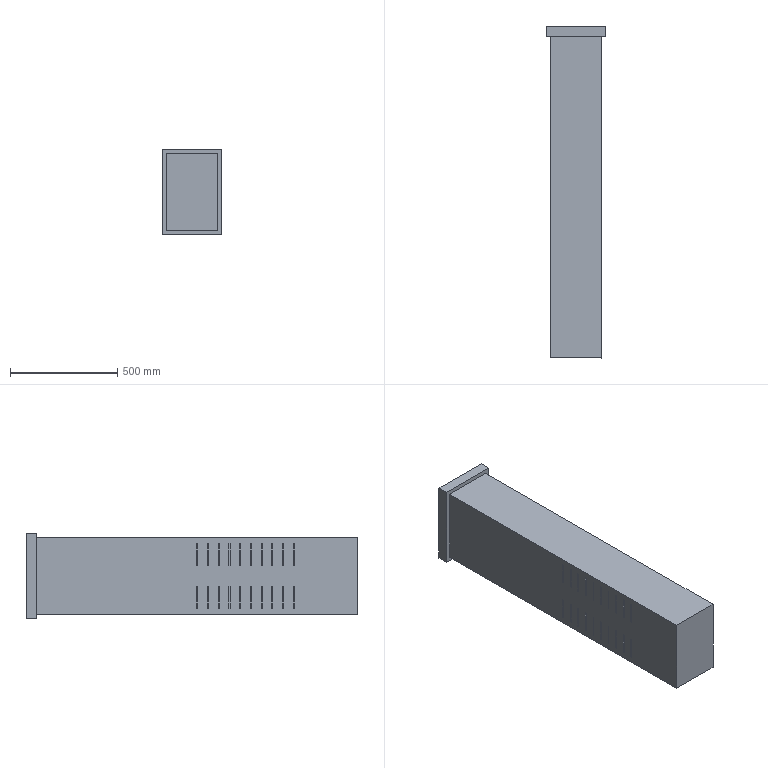Component | SolidWorks | LiftingAndOperatingMechanism-1_18-1 | 1 solid | 111 faces | box 280 x 1550 x 400 mm | volume 135150000 mm3 | plane 111
build123d program:
from build123d import *

# Parameters (mm, degrees)
SKETCH1_W           = 400
SKETCH1_H           = 280
BOSS_EXTRUDE1_DEPTH = 50
SKETCH2_W           = 360
SKETCH2_H           = 240
BOSS_EXTRUDE2_DEPTH = 1500
SKETCH3_W           = 100
SKETCH3_H           = 5
CUT_EXTRUDE1_DEPTH  = 5


with BuildPart() as part:
    # Sketch1 → Boss-Extrude1 (new body)
    with BuildSketch(Plane(origin=(0, 0, 0), x_dir=(1, 0, 0), z_dir=(0, 1, 0))):
        Rectangle(SKETCH1_W, SKETCH1_H)
    extrude(amount=BOSS_EXTRUDE1_DEPTH)

    # Sketch2 → Boss-Extrude2 (add)
    with BuildSketch(Plane(origin=(0, 50, 0), x_dir=(1, 0, 0), z_dir=(0, 1, 0))):
        Rectangle(SKETCH2_W, SKETCH2_H)
    extrude(amount=BOSS_EXTRUDE2_DEPTH)

    # Sketch3 → Cut-Extrude1 (cut)
    with BuildSketch(Plane.XY.offset(120)):
        with Locations((-100, 1250)):
            Rectangle(SKETCH3_W, SKETCH3_H)
        with Locations((100, 1250)):
            Rectangle(SKETCH3_W, SKETCH3_H)
        with Locations((-100, 1200)):
            Rectangle(SKETCH3_W, SKETCH3_H)
        with Locations((100, 1200)):
            Rectangle(SKETCH3_W, SKETCH3_H)
        with Locations((-100, 1150)):
            Rectangle(SKETCH3_W, SKETCH3_H)
        with Locations((100, 1150)):
            Rectangle(SKETCH3_W, SKETCH3_H)
        with Locations((-100, 1100)):
            Rectangle(SKETCH3_W, SKETCH3_H)
        with Locations((100, 1100)):
            Rectangle(SKETCH3_W, SKETCH3_H)
        with Locations((-100, 1050)):
            Rectangle(SKETCH3_W, SKETCH3_H)
        with Locations((100, 1050)):
            Rectangle(SKETCH3_W, SKETCH3_H)
        with Locations((-100, 1000)):
            Rectangle(SKETCH3_W, SKETCH3_H)
        with Locations((100, 1000)):
            Rectangle(SKETCH3_W, SKETCH3_H)
        with Locations((-100, 950)):
            Rectangle(SKETCH3_W, SKETCH3_H)
        with Locations((100, 950)):
            Rectangle(SKETCH3_W, SKETCH3_H)
        with Locations((-100, 900)):
            Rectangle(SKETCH3_W, SKETCH3_H)
        with Locations((100, 900)):
            Rectangle(SKETCH3_W, SKETCH3_H)
        with Locations((-100, 850)):
            Rectangle(SKETCH3_W, SKETCH3_H)
        with Locations((100, 850)):
            Rectangle(SKETCH3_W, SKETCH3_H)
        with Locations((-100, 800)):
            Rectangle(SKETCH3_W, SKETCH3_H)
        with Locations((100, 800)):
            Rectangle(SKETCH3_W, SKETCH3_H)
    extrude(amount=-CUT_EXTRUDE1_DEPTH, mode=Mode.SUBTRACT)


solid = part.part

# Placed as in the assembly
solid = solid.moved(Location((-418.963, 12438.918, 5832.153), (180, -90, 0)))